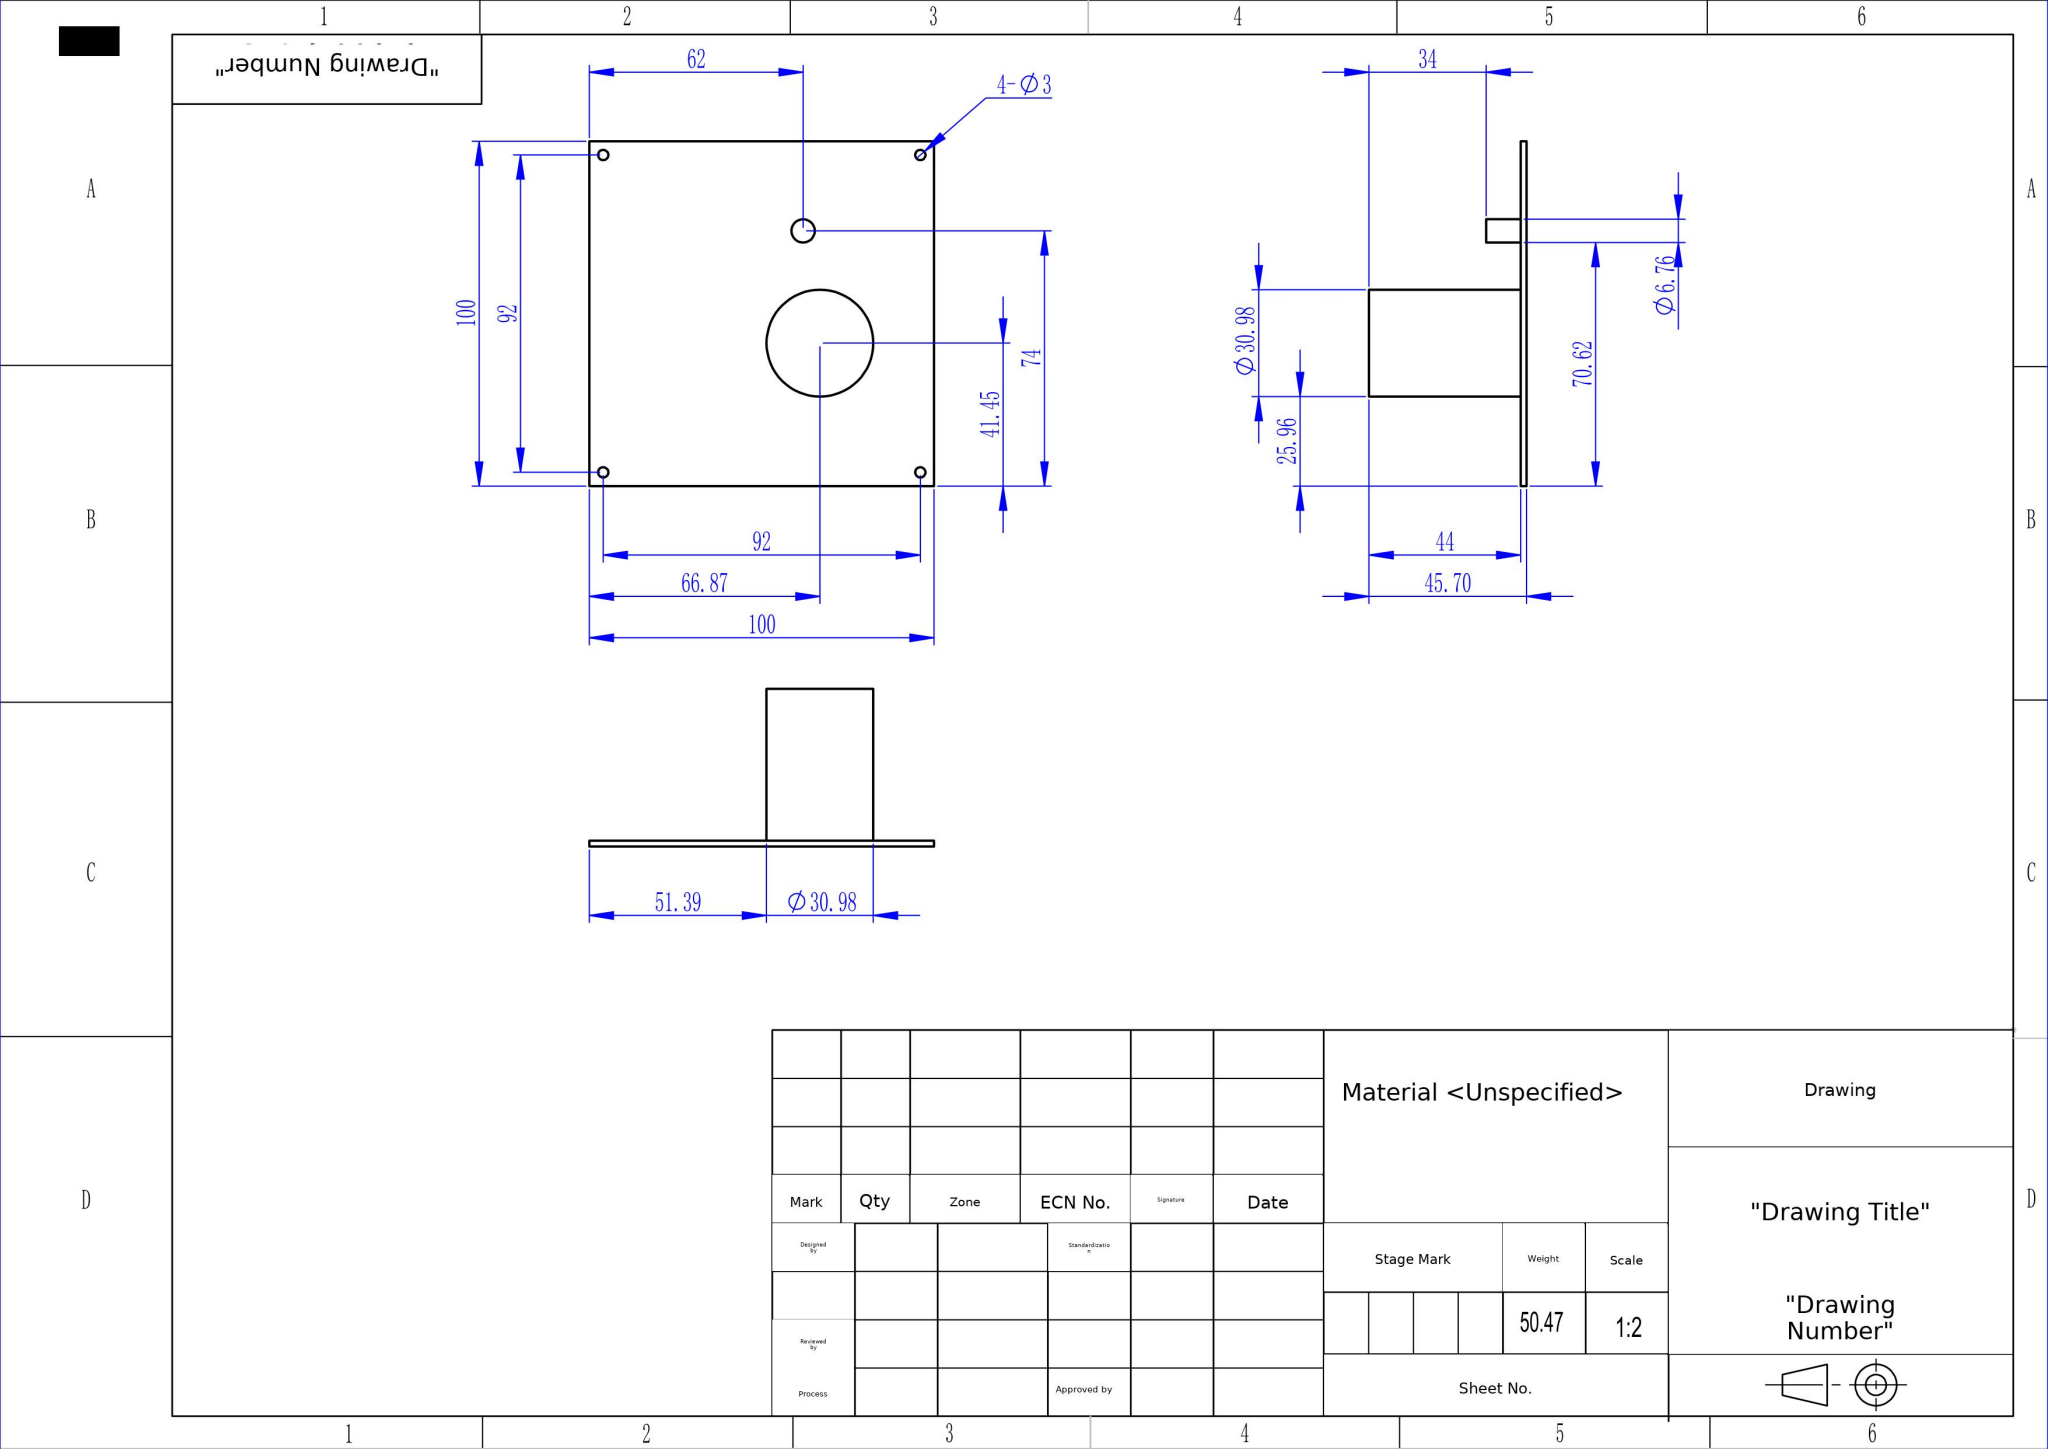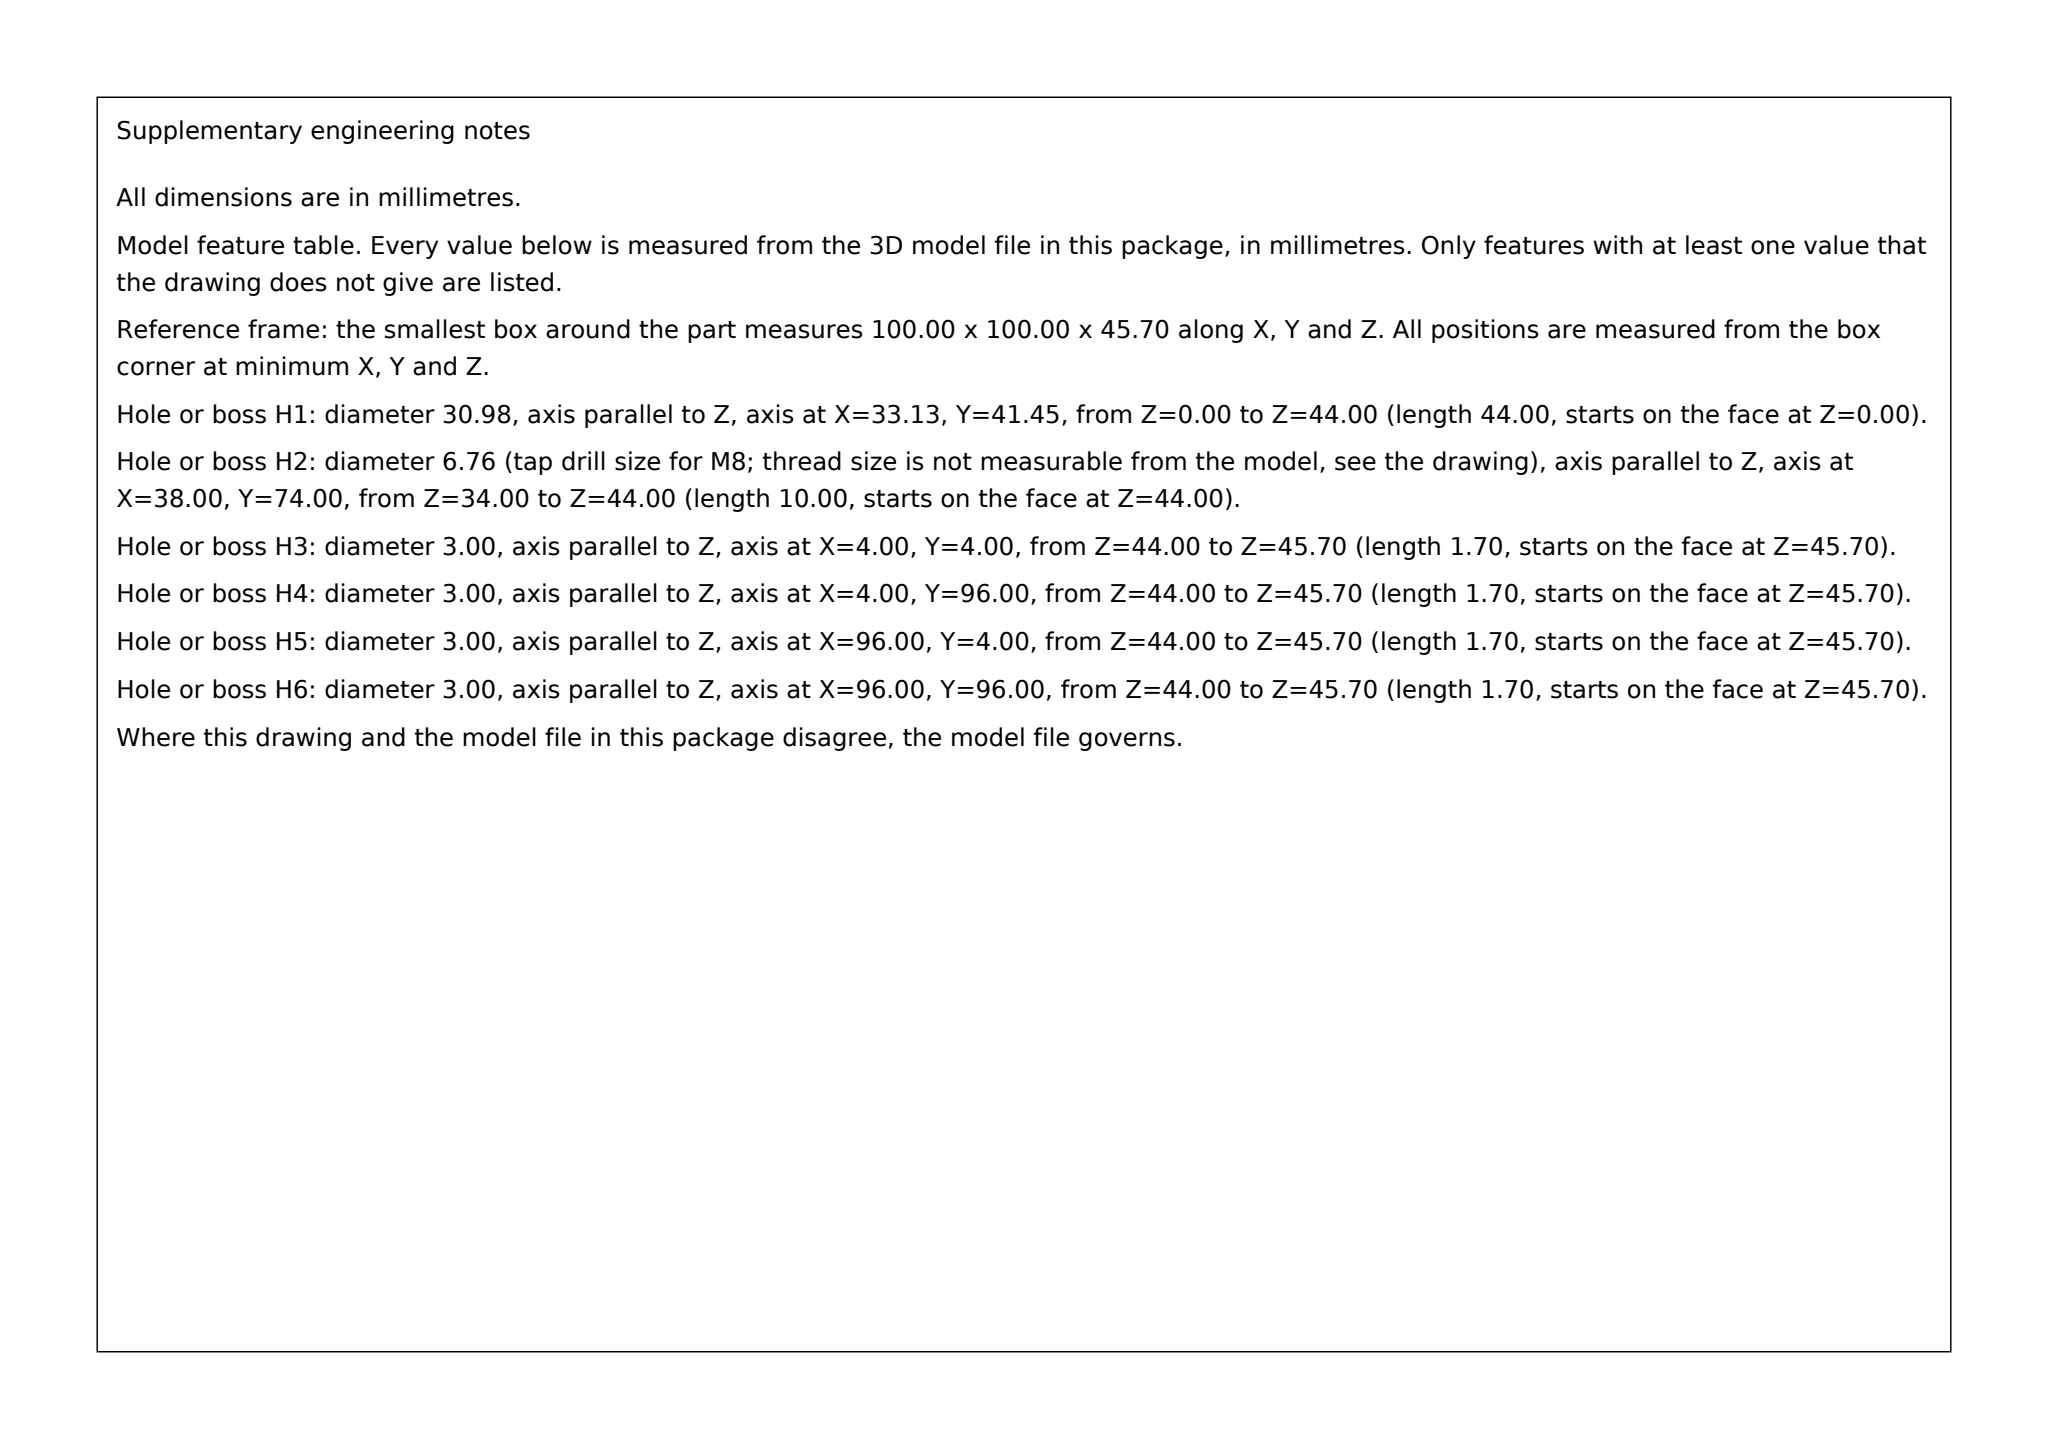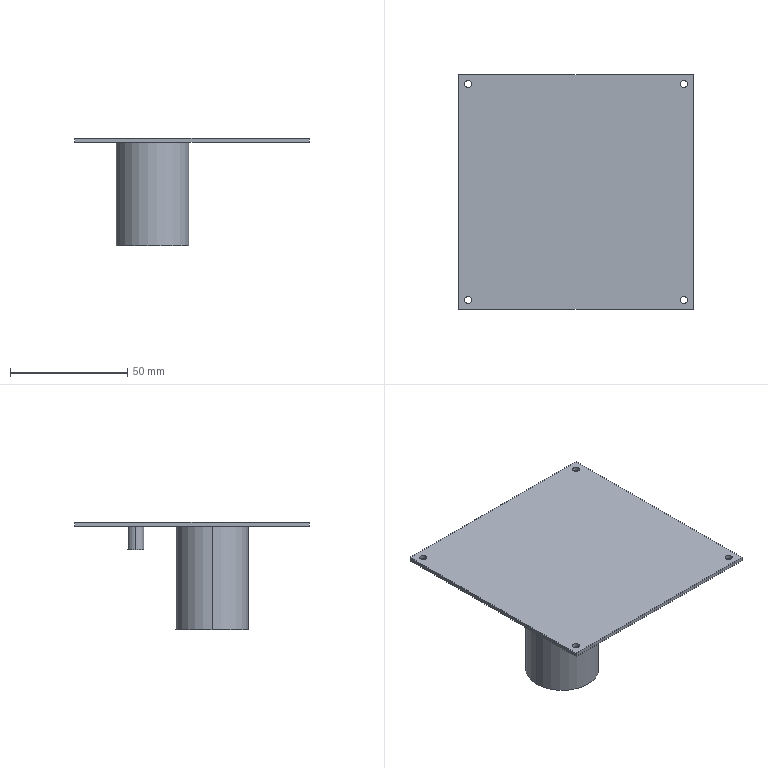Part | SolidWorks | mm | 1 solid | 20 faces | box 100 x 100 x 45.7 mm | volume 50474 mm3 | cylinder 12 | plane 8 | commonest cylinder face diameters 3 x8 6.758 x2 30.978 x2
build123d program:
from build123d import *

# Parameters (mm, degrees)
SKETCH1_W           = 100
SKETCH1_H           = 100
SKETCH1_R           = 1.5
BOSS_EXTRUDE1_DEPTH = 1.7
SKETCH3_R           = 15.489
BOSS_EXTRUDE3_DEPTH = 44
SKETCH5_R           = 3.379
BOSS_EXTRUDE4_DEPTH = 10


with BuildPart() as part:
    # Sketch1 → Boss-Extrude1 (new body)
    with BuildSketch(Plane.XY):
        Rectangle(SKETCH1_W, SKETCH1_H)
        with Locations((46, -46)):
            Circle(SKETCH1_R, mode=Mode.SUBTRACT)
        with Locations((46, 46)):
            Circle(SKETCH1_R, mode=Mode.SUBTRACT)
        with Locations((-46, 46)):
            Circle(SKETCH1_R, mode=Mode.SUBTRACT)
        with Locations((-46, -46)):
            Circle(SKETCH1_R, mode=Mode.SUBTRACT)
    extrude(amount=BOSS_EXTRUDE1_DEPTH)

    # Sketch3 → Boss-Extrude3 (add)
    with BuildSketch(Plane(origin=(0, 0, 0), x_dir=(-1, 0, 0), z_dir=(0, 0, -1))):
        with Locations((16.875, -8.549)):
            Circle(SKETCH3_R)
    extrude(amount=BOSS_EXTRUDE3_DEPTH)

    # Sketch5 → Boss-Extrude4 (add)
    with BuildSketch(Plane(origin=(0, 0, 0), x_dir=(-1, 0, 0), z_dir=(0, 0, -1))):
        with Locations((12, 24)):
            Circle(SKETCH5_R)
    extrude(amount=BOSS_EXTRUDE4_DEPTH)


solid = part.part
STEP:
#1=CARTESIAN_POINT('',(-15.379,24.,-10.));
#2=VERTEX_POINT('',#1);
#3=CARTESIAN_POINT('',(-8.621,24.,-10.));
#4=VERTEX_POINT('',#3);
#5=CARTESIAN_POINT('',(-12.,24.,-10.));
#6=DIRECTION('',(0.,0.,-1.));
#7=DIRECTION('',(-1.,0.,0.));
#8=AXIS2_PLACEMENT_3D('',#5,#6,#7);
#9=CIRCLE('',#8,3.379);
#10=EDGE_CURVE('',#2,#4,#9,.T.);
#11=ORIENTED_EDGE('',*,*,#10,.F.);
#12=CARTESIAN_POINT('',(-15.379,24.,0.));
#13=VERTEX_POINT('',#12);
#14=CARTESIAN_POINT('',(-15.379,24.,-10.));
#15=DIRECTION('',(0.,0.,1.));
#16=VECTOR('',#15,1000.);
#17=LINE('',#14,#16);
#18=EDGE_CURVE('',#2,#13,#17,.T.);
#19=ORIENTED_EDGE('',*,*,#18,.T.);
#20=CARTESIAN_POINT('',(-8.621,24.,0.));
#21=VERTEX_POINT('',#20);
#22=CARTESIAN_POINT('',(-12.,24.,0.));
#23=DIRECTION('',(0.,0.,-1.));
#24=DIRECTION('',(-1.,0.,0.));
#25=AXIS2_PLACEMENT_3D('',#22,#23,#24);
#26=CIRCLE('',#25,3.379);
#27=EDGE_CURVE('',#13,#21,#26,.T.);
#28=ORIENTED_EDGE('',*,*,#27,.T.);
#29=CARTESIAN_POINT('',(-8.621,24.,-10.));
#30=DIRECTION('',(0.,0.,1.));
#31=VECTOR('',#30,1000.);
#32=LINE('',#29,#31);
#33=EDGE_CURVE('',#4,#21,#32,.T.);
#34=ORIENTED_EDGE('',*,*,#33,.F.);
#35=EDGE_LOOP('',(#11,#19,#28,#34));
#36=FACE_OUTER_BOUND('',#35,.T.);
#37=CARTESIAN_POINT('',(-12.,24.,-10.));
#38=DIRECTION('',(0.,0.,1.));
#39=DIRECTION('',(1.,0.,0.));
#40=AXIS2_PLACEMENT_3D('',#37,#38,#39);
#41=CYLINDRICAL_SURFACE('',#40,3.379);
#42=ADVANCED_FACE('',(#36),#41,.T.);
#43=CARTESIAN_POINT('',(-32.364,-8.549,-44.));
#44=VERTEX_POINT('',#43);
#45=CARTESIAN_POINT('',(-1.386,-8.549,-44.));
#46=VERTEX_POINT('',#45);
#47=CARTESIAN_POINT('',(-16.875,-8.549,-44.));
#48=DIRECTION('',(0.,0.,-1.));
#49=DIRECTION('',(-1.,0.,0.));
#50=AXIS2_PLACEMENT_3D('',#47,#48,#49);
#51=CIRCLE('',#50,15.489);
#52=EDGE_CURVE('',#44,#46,#51,.T.);
#53=ORIENTED_EDGE('',*,*,#52,.F.);
#54=CARTESIAN_POINT('',(-32.364,-8.549,0.));
#55=VERTEX_POINT('',#54);
#56=CARTESIAN_POINT('',(-32.364,-8.549,-44.));
#57=DIRECTION('',(0.,0.,1.));
#58=VECTOR('',#57,1000.);
#59=LINE('',#56,#58);
#60=EDGE_CURVE('',#44,#55,#59,.T.);
#61=ORIENTED_EDGE('',*,*,#60,.T.);
#62=CARTESIAN_POINT('',(-1.386,-8.549,0.));
#63=VERTEX_POINT('',#62);
#64=CARTESIAN_POINT('',(-16.875,-8.549,0.));
#65=DIRECTION('',(0.,0.,-1.));
#66=DIRECTION('',(-1.,0.,0.));
#67=AXIS2_PLACEMENT_3D('',#64,#65,#66);
#68=CIRCLE('',#67,15.489);
#69=EDGE_CURVE('',#55,#63,#68,.T.);
#70=ORIENTED_EDGE('',*,*,#69,.T.);
#71=CARTESIAN_POINT('',(-1.386,-8.549,-44.));
#72=DIRECTION('',(0.,0.,1.));
#73=VECTOR('',#72,1000.);
#74=LINE('',#71,#73);
#75=EDGE_CURVE('',#46,#63,#74,.T.);
#76=ORIENTED_EDGE('',*,*,#75,.F.);
#77=EDGE_LOOP('',(#53,#61,#70,#76));
#78=FACE_OUTER_BOUND('',#77,.T.);
#79=CARTESIAN_POINT('',(-16.875,-8.549,-44.));
#80=DIRECTION('',(0.,0.,1.));
#81=DIRECTION('',(1.,0.,0.));
#82=AXIS2_PLACEMENT_3D('',#79,#80,#81);
#83=CYLINDRICAL_SURFACE('',#82,15.489);
#84=ADVANCED_FACE('',(#78),#83,.T.);
#85=CARTESIAN_POINT('',(-47.5,-46.,1.7));
#86=VERTEX_POINT('',#85);
#87=CARTESIAN_POINT('',(-44.5,-46.,1.7));
#88=VERTEX_POINT('',#87);
#89=CARTESIAN_POINT('',(-46.,-46.,1.7));
#90=DIRECTION('',(0.,0.,1.));
#91=DIRECTION('',(1.,0.,0.));
#92=AXIS2_PLACEMENT_3D('',#89,#90,#91);
#93=CIRCLE('',#92,1.5);
#94=EDGE_CURVE('',#86,#88,#93,.T.);
#95=ORIENTED_EDGE('',*,*,#94,.T.);
#96=CARTESIAN_POINT('',(-44.5,-46.,0.));
#97=VERTEX_POINT('',#96);
#98=CARTESIAN_POINT('',(-44.5,-46.,1.7));
#99=DIRECTION('',(0.,0.,-1.));
#100=VECTOR('',#99,1000.);
#101=LINE('',#98,#100);
#102=EDGE_CURVE('',#88,#97,#101,.T.);
#103=ORIENTED_EDGE('',*,*,#102,.T.);
#104=CARTESIAN_POINT('',(-47.5,-46.,0.));
#105=VERTEX_POINT('',#104);
#106=CARTESIAN_POINT('',(-46.,-46.,0.));
#107=DIRECTION('',(0.,0.,1.));
#108=DIRECTION('',(1.,0.,0.));
#109=AXIS2_PLACEMENT_3D('',#106,#107,#108);
#110=CIRCLE('',#109,1.5);
#111=EDGE_CURVE('',#105,#97,#110,.T.);
#112=ORIENTED_EDGE('',*,*,#111,.F.);
#113=CARTESIAN_POINT('',(-47.5,-46.,1.7));
#114=DIRECTION('',(0.,0.,-1.));
#115=VECTOR('',#114,1000.);
#116=LINE('',#113,#115);
#117=EDGE_CURVE('',#86,#105,#116,.T.);
#118=ORIENTED_EDGE('',*,*,#117,.F.);
#119=EDGE_LOOP('',(#95,#103,#112,#118));
#120=FACE_OUTER_BOUND('',#119,.T.);
#121=CARTESIAN_POINT('',(-46.,-46.,1.7));
#122=DIRECTION('',(0.,0.,-1.));
#123=DIRECTION('',(-1.,0.,0.));
#124=AXIS2_PLACEMENT_3D('',#121,#122,#123);
#125=CYLINDRICAL_SURFACE('',#124,1.5);
#126=ADVANCED_FACE('',(#120),#125,.F.);
#127=CARTESIAN_POINT('',(-47.5,46.,1.7));
#128=VERTEX_POINT('',#127);
#129=CARTESIAN_POINT('',(-44.5,46.,1.7));
#130=VERTEX_POINT('',#129);
#131=CARTESIAN_POINT('',(-46.,46.,1.7));
#132=DIRECTION('',(0.,0.,1.));
#133=DIRECTION('',(1.,0.,0.));
#134=AXIS2_PLACEMENT_3D('',#131,#132,#133);
#135=CIRCLE('',#134,1.5);
#136=EDGE_CURVE('',#128,#130,#135,.T.);
#137=ORIENTED_EDGE('',*,*,#136,.T.);
#138=CARTESIAN_POINT('',(-44.5,46.,0.));
#139=VERTEX_POINT('',#138);
#140=CARTESIAN_POINT('',(-44.5,46.,1.7));
#141=DIRECTION('',(0.,0.,-1.));
#142=VECTOR('',#141,1000.);
#143=LINE('',#140,#142);
#144=EDGE_CURVE('',#130,#139,#143,.T.);
#145=ORIENTED_EDGE('',*,*,#144,.T.);
#146=CARTESIAN_POINT('',(-47.5,46.,0.));
#147=VERTEX_POINT('',#146);
#148=CARTESIAN_POINT('',(-46.,46.,0.));
#149=DIRECTION('',(0.,0.,1.));
#150=DIRECTION('',(1.,0.,0.));
#151=AXIS2_PLACEMENT_3D('',#148,#149,#150);
#152=CIRCLE('',#151,1.5);
#153=EDGE_CURVE('',#147,#139,#152,.T.);
#154=ORIENTED_EDGE('',*,*,#153,.F.);
#155=CARTESIAN_POINT('',(-47.5,46.,1.7));
#156=DIRECTION('',(0.,0.,-1.));
#157=VECTOR('',#156,1000.);
#158=LINE('',#155,#157);
#159=EDGE_CURVE('',#128,#147,#158,.T.);
#160=ORIENTED_EDGE('',*,*,#159,.F.);
#161=EDGE_LOOP('',(#137,#145,#154,#160));
#162=FACE_OUTER_BOUND('',#161,.T.);
#163=CARTESIAN_POINT('',(-46.,46.,1.7));
#164=DIRECTION('',(0.,0.,-1.));
#165=DIRECTION('',(-1.,0.,0.));
#166=AXIS2_PLACEMENT_3D('',#163,#164,#165);
#167=CYLINDRICAL_SURFACE('',#166,1.5);
#168=ADVANCED_FACE('',(#162),#167,.F.);
#169=CARTESIAN_POINT('',(44.5,46.,1.7));
#170=VERTEX_POINT('',#169);
#171=CARTESIAN_POINT('',(47.5,46.,1.7));
#172=VERTEX_POINT('',#171);
#173=CARTESIAN_POINT('',(46.,46.,1.7));
#174=DIRECTION('',(0.,0.,1.));
#175=DIRECTION('',(1.,0.,0.));
#176=AXIS2_PLACEMENT_3D('',#173,#174,#175);
#177=CIRCLE('',#176,1.5);
#178=EDGE_CURVE('',#170,#172,#177,.T.);
#179=ORIENTED_EDGE('',*,*,#178,.T.);
#180=CARTESIAN_POINT('',(47.5,46.,0.));
#181=VERTEX_POINT('',#180);
#182=CARTESIAN_POINT('',(47.5,46.,1.7));
#183=DIRECTION('',(0.,0.,-1.));
#184=VECTOR('',#183,1000.);
#185=LINE('',#182,#184);
#186=EDGE_CURVE('',#172,#181,#185,.T.);
#187=ORIENTED_EDGE('',*,*,#186,.T.);
#188=CARTESIAN_POINT('',(44.5,46.,0.));
#189=VERTEX_POINT('',#188);
#190=CARTESIAN_POINT('',(46.,46.,0.));
#191=DIRECTION('',(0.,0.,1.));
#192=DIRECTION('',(1.,0.,0.));
#193=AXIS2_PLACEMENT_3D('',#190,#191,#192);
#194=CIRCLE('',#193,1.5);
#195=EDGE_CURVE('',#189,#181,#194,.T.);
#196=ORIENTED_EDGE('',*,*,#195,.F.);
#197=CARTESIAN_POINT('',(44.5,46.,1.7));
#198=DIRECTION('',(0.,0.,-1.));
#199=VECTOR('',#198,1000.);
#200=LINE('',#197,#199);
#201=EDGE_CURVE('',#170,#189,#200,.T.);
#202=ORIENTED_EDGE('',*,*,#201,.F.);
#203=EDGE_LOOP('',(#179,#187,#196,#202));
#204=FACE_OUTER_BOUND('',#203,.T.);
#205=CARTESIAN_POINT('',(46.,46.,1.7));
#206=DIRECTION('',(0.,0.,-1.));
#207=DIRECTION('',(-1.,0.,0.));
#208=AXIS2_PLACEMENT_3D('',#205,#206,#207);
#209=CYLINDRICAL_SURFACE('',#208,1.5);
#210=ADVANCED_FACE('',(#204),#209,.F.);
#211=CARTESIAN_POINT('',(44.5,-46.,1.7));
#212=VERTEX_POINT('',#211);
#213=CARTESIAN_POINT('',(47.5,-46.,1.7));
#214=VERTEX_POINT('',#213);
#215=CARTESIAN_POINT('',(46.,-46.,1.7));
#216=DIRECTION('',(0.,0.,1.));
#217=DIRECTION('',(1.,0.,0.));
#218=AXIS2_PLACEMENT_3D('',#215,#216,#217);
#219=CIRCLE('',#218,1.5);
#220=EDGE_CURVE('',#212,#214,#219,.T.);
#221=ORIENTED_EDGE('',*,*,#220,.T.);
#222=CARTESIAN_POINT('',(47.5,-46.,0.));
#223=VERTEX_POINT('',#222);
#224=CARTESIAN_POINT('',(47.5,-46.,1.7));
#225=DIRECTION('',(0.,0.,-1.));
#226=VECTOR('',#225,1000.);
#227=LINE('',#224,#226);
#228=EDGE_CURVE('',#214,#223,#227,.T.);
#229=ORIENTED_EDGE('',*,*,#228,.T.);
#230=CARTESIAN_POINT('',(44.5,-46.,0.));
#231=VERTEX_POINT('',#230);
#232=CARTESIAN_POINT('',(46.,-46.,0.));
#233=DIRECTION('',(0.,0.,1.));
#234=DIRECTION('',(1.,0.,0.));
#235=AXIS2_PLACEMENT_3D('',#232,#233,#234);
#236=CIRCLE('',#235,1.5);
#237=EDGE_CURVE('',#231,#223,#236,.T.);
#238=ORIENTED_EDGE('',*,*,#237,.F.);
#239=CARTESIAN_POINT('',(44.5,-46.,1.7));
#240=DIRECTION('',(0.,0.,-1.));
#241=VECTOR('',#240,1000.);
#242=LINE('',#239,#241);
#243=EDGE_CURVE('',#212,#231,#242,.T.);
#244=ORIENTED_EDGE('',*,*,#243,.F.);
#245=EDGE_LOOP('',(#221,#229,#238,#244));
#246=FACE_OUTER_BOUND('',#245,.T.);
#247=CARTESIAN_POINT('',(46.,-46.,1.7));
#248=DIRECTION('',(0.,0.,-1.));
#249=DIRECTION('',(-1.,0.,0.));
#250=AXIS2_PLACEMENT_3D('',#247,#248,#249);
#251=CYLINDRICAL_SURFACE('',#250,1.5);
#252=ADVANCED_FACE('',(#246),#251,.F.);
#253=CARTESIAN_POINT('',(50.,-50.,1.7));
#254=VERTEX_POINT('',#253);
#255=CARTESIAN_POINT('',(50.,50.,1.7));
#256=VERTEX_POINT('',#255);
#257=CARTESIAN_POINT('',(50.,-50.,1.7));
#258=DIRECTION('',(0.,1.,0.));
#259=VECTOR('',#258,1000.);
#260=LINE('',#257,#259);
#261=EDGE_CURVE('',#254,#256,#260,.T.);
#262=ORIENTED_EDGE('',*,*,#261,.T.);
#263=CARTESIAN_POINT('',(-50.,50.,1.7));
#264=VERTEX_POINT('',#263);
#265=CARTESIAN_POINT('',(-50.,50.,1.7));
#266=DIRECTION('',(-1.,0.,0.));
#267=VECTOR('',#266,1000.);
#268=LINE('',#265,#267);
#269=EDGE_CURVE('',#256,#264,#268,.T.);
#270=ORIENTED_EDGE('',*,*,#269,.T.);
#271=CARTESIAN_POINT('',(-50.,-50.,1.7));
#272=VERTEX_POINT('',#271);
#273=CARTESIAN_POINT('',(-50.,-50.,1.7));
#274=DIRECTION('',(0.,-1.,0.));
#275=VECTOR('',#274,1000.);
#276=LINE('',#273,#275);
#277=EDGE_CURVE('',#264,#272,#276,.T.);
#278=ORIENTED_EDGE('',*,*,#277,.T.);
#279=CARTESIAN_POINT('',(-50.,-50.,1.7));
#280=DIRECTION('',(1.,0.,0.));
#281=VECTOR('',#280,1000.);
#282=LINE('',#279,#281);
#283=EDGE_CURVE('',#272,#254,#282,.T.);
#284=ORIENTED_EDGE('',*,*,#283,.T.);
#285=EDGE_LOOP('',(#262,#270,#278,#284));
#286=FACE_OUTER_BOUND('',#285,.T.);
#287=ORIENTED_EDGE('',*,*,#220,.F.);
#288=CARTESIAN_POINT('',(46.,-46.,1.7));
#289=DIRECTION('',(0.,0.,1.));
#290=DIRECTION('',(1.,0.,0.));
#291=AXIS2_PLACEMENT_3D('',#288,#289,#290);
#292=CIRCLE('',#291,1.5);
#293=EDGE_CURVE('',#214,#212,#292,.T.);
#294=ORIENTED_EDGE('',*,*,#293,.F.);
#295=EDGE_LOOP('',(#287,#294));
#296=FACE_BOUND('',#295,.T.);
#297=ORIENTED_EDGE('',*,*,#178,.F.);
#298=CARTESIAN_POINT('',(46.,46.,1.7));
#299=DIRECTION('',(0.,0.,1.));
#300=DIRECTION('',(1.,0.,0.));
#301=AXIS2_PLACEMENT_3D('',#298,#299,#300);
#302=CIRCLE('',#301,1.5);
#303=EDGE_CURVE('',#172,#170,#302,.T.);
#304=ORIENTED_EDGE('',*,*,#303,.F.);
#305=EDGE_LOOP('',(#297,#304));
#306=FACE_BOUND('',#305,.T.);
#307=ORIENTED_EDGE('',*,*,#136,.F.);
#308=CARTESIAN_POINT('',(-46.,46.,1.7));
#309=DIRECTION('',(0.,0.,1.));
#310=DIRECTION('',(1.,0.,0.));
#311=AXIS2_PLACEMENT_3D('',#308,#309,#310);
#312=CIRCLE('',#311,1.5);
#313=EDGE_CURVE('',#130,#128,#312,.T.);
#314=ORIENTED_EDGE('',*,*,#313,.F.);
#315=EDGE_LOOP('',(#307,#314));
#316=FACE_BOUND('',#315,.T.);
#317=ORIENTED_EDGE('',*,*,#94,.F.);
#318=CARTESIAN_POINT('',(-46.,-46.,1.7));
#319=DIRECTION('',(0.,0.,1.));
#320=DIRECTION('',(1.,0.,0.));
#321=AXIS2_PLACEMENT_3D('',#318,#319,#320);
#322=CIRCLE('',#321,1.5);
#323=EDGE_CURVE('',#88,#86,#322,.T.);
#324=ORIENTED_EDGE('',*,*,#323,.F.);
#325=EDGE_LOOP('',(#317,#324));
#326=FACE_BOUND('',#325,.T.);
#327=CARTESIAN_POINT('',(0.,0.,1.7));
#328=DIRECTION('',(0.,0.,-1.));
#329=DIRECTION('',(-1.,0.,0.));
#330=AXIS2_PLACEMENT_3D('',#327,#328,#329);
#331=PLANE('',#330);
#332=ADVANCED_FACE('',(#286,#296,#306,#316,#326),#331,.F.);
#333=CARTESIAN_POINT('',(-12.,24.,0.));
#334=DIRECTION('',(0.,0.,-1.));
#335=DIRECTION('',(-1.,0.,0.));
#336=AXIS2_PLACEMENT_3D('',#333,#334,#335);
#337=CIRCLE('',#336,3.379);
#338=EDGE_CURVE('',#21,#13,#337,.T.);
#339=ORIENTED_EDGE('',*,*,#338,.F.);
#340=ORIENTED_EDGE('',*,*,#27,.F.);
#341=EDGE_LOOP('',(#339,#340));
#342=FACE_BOUND('',#341,.T.);
#343=CARTESIAN_POINT('',(-16.875,-8.549,0.));
#344=DIRECTION('',(0.,0.,-1.));
#345=DIRECTION('',(-1.,0.,0.));
#346=AXIS2_PLACEMENT_3D('',#343,#344,#345);
#347=CIRCLE('',#346,15.489);
#348=EDGE_CURVE('',#63,#55,#347,.T.);
#349=ORIENTED_EDGE('',*,*,#348,.F.);
#350=ORIENTED_EDGE('',*,*,#69,.F.);
#351=EDGE_LOOP('',(#349,#350));
#352=FACE_BOUND('',#351,.T.);
#353=ORIENTED_EDGE('',*,*,#153,.T.);
#354=CARTESIAN_POINT('',(-46.,46.,0.));
#355=DIRECTION('',(0.,0.,1.));
#356=DIRECTION('',(1.,0.,0.));
#357=AXIS2_PLACEMENT_3D('',#354,#355,#356);
#358=CIRCLE('',#357,1.5);
#359=EDGE_CURVE('',#139,#147,#358,.T.);
#360=ORIENTED_EDGE('',*,*,#359,.T.);
#361=EDGE_LOOP('',(#353,#360));
#362=FACE_BOUND('',#361,.T.);
#363=ORIENTED_EDGE('',*,*,#237,.T.);
#364=CARTESIAN_POINT('',(46.,-46.,0.));
#365=DIRECTION('',(0.,0.,1.));
#366=DIRECTION('',(1.,0.,0.));
#367=AXIS2_PLACEMENT_3D('',#364,#365,#366);
#368=CIRCLE('',#367,1.5);
#369=EDGE_CURVE('',#223,#231,#368,.T.);
#370=ORIENTED_EDGE('',*,*,#369,.T.);
#371=EDGE_LOOP('',(#363,#370));
#372=FACE_BOUND('',#371,.T.);
#373=CARTESIAN_POINT('',(50.,-50.,0.));
#374=VERTEX_POINT('',#373);
#375=CARTESIAN_POINT('',(50.,50.,0.));
#376=VERTEX_POINT('',#375);
#377=CARTESIAN_POINT('',(50.,-50.,0.));
#378=DIRECTION('',(0.,1.,0.));
#379=VECTOR('',#378,1000.);
#380=LINE('',#377,#379);
#381=EDGE_CURVE('',#374,#376,#380,.T.);
#382=ORIENTED_EDGE('',*,*,#381,.F.);
#383=CARTESIAN_POINT('',(-50.,-50.,0.));
#384=VERTEX_POINT('',#383);
#385=CARTESIAN_POINT('',(-50.,-50.,0.));
#386=DIRECTION('',(1.,0.,0.));
#387=VECTOR('',#386,1000.);
#388=LINE('',#385,#387);
#389=EDGE_CURVE('',#384,#374,#388,.T.);
#390=ORIENTED_EDGE('',*,*,#389,.F.);
#391=CARTESIAN_POINT('',(-50.,50.,0.));
#392=VERTEX_POINT('',#391);
#393=CARTESIAN_POINT('',(-50.,-50.,0.));
#394=DIRECTION('',(0.,-1.,0.));
#395=VECTOR('',#394,1000.);
#396=LINE('',#393,#395);
#397=EDGE_CURVE('',#392,#384,#396,.T.);
#398=ORIENTED_EDGE('',*,*,#397,.F.);
#399=CARTESIAN_POINT('',(-50.,50.,0.));
#400=DIRECTION('',(-1.,0.,0.));
#401=VECTOR('',#400,1000.);
#402=LINE('',#399,#401);
#403=EDGE_CURVE('',#376,#392,#402,.T.);
#404=ORIENTED_EDGE('',*,*,#403,.F.);
#405=EDGE_LOOP('',(#382,#390,#398,#404));
#406=FACE_OUTER_BOUND('',#405,.T.);
#407=ORIENTED_EDGE('',*,*,#195,.T.);
#408=CARTESIAN_POINT('',(46.,46.,0.));
#409=DIRECTION('',(0.,0.,1.));
#410=DIRECTION('',(1.,0.,0.));
#411=AXIS2_PLACEMENT_3D('',#408,#409,#410);
#412=CIRCLE('',#411,1.5);
#413=EDGE_CURVE('',#181,#189,#412,.T.);
#414=ORIENTED_EDGE('',*,*,#413,.T.);
#415=EDGE_LOOP('',(#407,#414));
#416=FACE_BOUND('',#415,.T.);
#417=ORIENTED_EDGE('',*,*,#111,.T.);
#418=CARTESIAN_POINT('',(-46.,-46.,0.));
#419=DIRECTION('',(0.,0.,1.));
#420=DIRECTION('',(1.,0.,0.));
#421=AXIS2_PLACEMENT_3D('',#418,#419,#420);
#422=CIRCLE('',#421,1.5);
#423=EDGE_CURVE('',#97,#105,#422,.T.);
#424=ORIENTED_EDGE('',*,*,#423,.T.);
#425=EDGE_LOOP('',(#417,#424));
#426=FACE_BOUND('',#425,.T.);
#427=CARTESIAN_POINT('',(0.,0.,0.));
#428=DIRECTION('',(0.,0.,-1.));
#429=DIRECTION('',(-1.,0.,0.));
#430=AXIS2_PLACEMENT_3D('',#427,#428,#429);
#431=PLANE('',#430);
#432=ADVANCED_FACE('',(#342,#352,#362,#372,#406,#416,#426),#431,.T.);
#433=ORIENTED_EDGE('',*,*,#381,.T.);
#434=CARTESIAN_POINT('',(50.,50.,1.7));
#435=DIRECTION('',(0.,0.,-1.));
#436=VECTOR('',#435,1000.);
#437=LINE('',#434,#436);
#438=EDGE_CURVE('',#256,#376,#437,.T.);
#439=ORIENTED_EDGE('',*,*,#438,.F.);
#440=ORIENTED_EDGE('',*,*,#261,.F.);
#441=CARTESIAN_POINT('',(50.,-50.,1.7));
#442=DIRECTION('',(0.,0.,-1.));
#443=VECTOR('',#442,1000.);
#444=LINE('',#441,#443);
#445=EDGE_CURVE('',#254,#374,#444,.T.);
#446=ORIENTED_EDGE('',*,*,#445,.T.);
#447=EDGE_LOOP('',(#433,#439,#440,#446));
#448=FACE_OUTER_BOUND('',#447,.T.);
#449=CARTESIAN_POINT('',(50.,-50.,1.7));
#450=DIRECTION('',(-1.,0.,0.));
#451=DIRECTION('',(0.,0.,1.));
#452=AXIS2_PLACEMENT_3D('',#449,#450,#451);
#453=PLANE('',#452);
#454=ADVANCED_FACE('',(#448),#453,.F.);
#455=ORIENTED_EDGE('',*,*,#403,.T.);
#456=CARTESIAN_POINT('',(-50.,50.,1.7));
#457=DIRECTION('',(0.,0.,-1.));
#458=VECTOR('',#457,1000.);
#459=LINE('',#456,#458);
#460=EDGE_CURVE('',#264,#392,#459,.T.);
#461=ORIENTED_EDGE('',*,*,#460,.F.);
#462=ORIENTED_EDGE('',*,*,#269,.F.);
#463=ORIENTED_EDGE('',*,*,#438,.T.);
#464=EDGE_LOOP('',(#455,#461,#462,#463));
#465=FACE_OUTER_BOUND('',#464,.T.);
#466=CARTESIAN_POINT('',(-50.,50.,1.7));
#467=DIRECTION('',(0.,-1.,0.));
#468=DIRECTION('',(0.,0.,-1.));
#469=AXIS2_PLACEMENT_3D('',#466,#467,#468);
#470=PLANE('',#469);
#471=ADVANCED_FACE('',(#465),#470,.F.);
#472=ORIENTED_EDGE('',*,*,#397,.T.);
#473=CARTESIAN_POINT('',(-50.,-50.,1.7));
#474=DIRECTION('',(0.,0.,-1.));
#475=VECTOR('',#474,1000.);
#476=LINE('',#473,#475);
#477=EDGE_CURVE('',#272,#384,#476,.T.);
#478=ORIENTED_EDGE('',*,*,#477,.F.);
#479=ORIENTED_EDGE('',*,*,#277,.F.);
#480=ORIENTED_EDGE('',*,*,#460,.T.);
#481=EDGE_LOOP('',(#472,#478,#479,#480));
#482=FACE_OUTER_BOUND('',#481,.T.);
#483=CARTESIAN_POINT('',(-50.,-50.,1.7));
#484=DIRECTION('',(1.,0.,0.));
#485=DIRECTION('',(0.,0.,-1.));
#486=AXIS2_PLACEMENT_3D('',#483,#484,#485);
#487=PLANE('',#486);
#488=ADVANCED_FACE('',(#482),#487,.F.);
#489=ORIENTED_EDGE('',*,*,#389,.T.);
#490=ORIENTED_EDGE('',*,*,#445,.F.);
#491=ORIENTED_EDGE('',*,*,#283,.F.);
#492=ORIENTED_EDGE('',*,*,#477,.T.);
#493=EDGE_LOOP('',(#489,#490,#491,#492));
#494=FACE_OUTER_BOUND('',#493,.T.);
#495=CARTESIAN_POINT('',(-50.,-50.,1.7));
#496=DIRECTION('',(0.,1.,0.));
#497=DIRECTION('',(0.,0.,1.));
#498=AXIS2_PLACEMENT_3D('',#495,#496,#497);
#499=PLANE('',#498);
#500=ADVANCED_FACE('',(#494),#499,.F.);
#501=ORIENTED_EDGE('',*,*,#228,.F.);
#502=ORIENTED_EDGE('',*,*,#293,.T.);
#503=ORIENTED_EDGE('',*,*,#243,.T.);
#504=ORIENTED_EDGE('',*,*,#369,.F.);
#505=EDGE_LOOP('',(#501,#502,#503,#504));
#506=FACE_OUTER_BOUND('',#505,.T.);
#507=CARTESIAN_POINT('',(46.,-46.,1.7));
#508=DIRECTION('',(0.,0.,-1.));
#509=DIRECTION('',(-1.,0.,0.));
#510=AXIS2_PLACEMENT_3D('',#507,#508,#509);
#511=CYLINDRICAL_SURFACE('',#510,1.5);
#512=ADVANCED_FACE('',(#506),#511,.F.);
#513=ORIENTED_EDGE('',*,*,#186,.F.);
#514=ORIENTED_EDGE('',*,*,#303,.T.);
#515=ORIENTED_EDGE('',*,*,#201,.T.);
#516=ORIENTED_EDGE('',*,*,#413,.F.);
#517=EDGE_LOOP('',(#513,#514,#515,#516));
#518=FACE_OUTER_BOUND('',#517,.T.);
#519=CARTESIAN_POINT('',(46.,46.,1.7));
#520=DIRECTION('',(0.,0.,-1.));
#521=DIRECTION('',(-1.,0.,0.));
#522=AXIS2_PLACEMENT_3D('',#519,#520,#521);
#523=CYLINDRICAL_SURFACE('',#522,1.5);
#524=ADVANCED_FACE('',(#518),#523,.F.);
#525=ORIENTED_EDGE('',*,*,#144,.F.);
#526=ORIENTED_EDGE('',*,*,#313,.T.);
#527=ORIENTED_EDGE('',*,*,#159,.T.);
#528=ORIENTED_EDGE('',*,*,#359,.F.);
#529=EDGE_LOOP('',(#525,#526,#527,#528));
#530=FACE_OUTER_BOUND('',#529,.T.);
#531=CARTESIAN_POINT('',(-46.,46.,1.7));
#532=DIRECTION('',(0.,0.,-1.));
#533=DIRECTION('',(-1.,0.,0.));
#534=AXIS2_PLACEMENT_3D('',#531,#532,#533);
#535=CYLINDRICAL_SURFACE('',#534,1.5);
#536=ADVANCED_FACE('',(#530),#535,.F.);
#537=ORIENTED_EDGE('',*,*,#102,.F.);
#538=ORIENTED_EDGE('',*,*,#323,.T.);
#539=ORIENTED_EDGE('',*,*,#117,.T.);
#540=ORIENTED_EDGE('',*,*,#423,.F.);
#541=EDGE_LOOP('',(#537,#538,#539,#540));
#542=FACE_OUTER_BOUND('',#541,.T.);
#543=CARTESIAN_POINT('',(-46.,-46.,1.7));
#544=DIRECTION('',(0.,0.,-1.));
#545=DIRECTION('',(-1.,0.,0.));
#546=AXIS2_PLACEMENT_3D('',#543,#544,#545);
#547=CYLINDRICAL_SURFACE('',#546,1.5);
#548=ADVANCED_FACE('',(#542),#547,.F.);
#549=ORIENTED_EDGE('',*,*,#60,.F.);
#550=CARTESIAN_POINT('',(-16.875,-8.549,-44.));
#551=DIRECTION('',(0.,0.,-1.));
#552=DIRECTION('',(-1.,0.,0.));
#553=AXIS2_PLACEMENT_3D('',#550,#551,#552);
#554=CIRCLE('',#553,15.489);
#555=EDGE_CURVE('',#46,#44,#554,.T.);
#556=ORIENTED_EDGE('',*,*,#555,.F.);
#557=ORIENTED_EDGE('',*,*,#75,.T.);
#558=ORIENTED_EDGE('',*,*,#348,.T.);
#559=EDGE_LOOP('',(#549,#556,#557,#558));
#560=FACE_OUTER_BOUND('',#559,.T.);
#561=CARTESIAN_POINT('',(-16.875,-8.549,-44.));
#562=DIRECTION('',(0.,0.,1.));
#563=DIRECTION('',(1.,0.,0.));
#564=AXIS2_PLACEMENT_3D('',#561,#562,#563);
#565=CYLINDRICAL_SURFACE('',#564,15.489);
#566=ADVANCED_FACE('',(#560),#565,.T.);
#567=ORIENTED_EDGE('',*,*,#555,.T.);
#568=ORIENTED_EDGE('',*,*,#52,.T.);
#569=EDGE_LOOP('',(#567,#568));
#570=FACE_OUTER_BOUND('',#569,.T.);
#571=CARTESIAN_POINT('',(-16.875,-8.549,-44.));
#572=DIRECTION('',(0.,0.,-1.));
#573=DIRECTION('',(-1.,0.,0.));
#574=AXIS2_PLACEMENT_3D('',#571,#572,#573);
#575=PLANE('',#574);
#576=ADVANCED_FACE('',(#570),#575,.T.);
#577=ORIENTED_EDGE('',*,*,#18,.F.);
#578=CARTESIAN_POINT('',(-12.,24.,-10.));
#579=DIRECTION('',(0.,0.,-1.));
#580=DIRECTION('',(-1.,0.,0.));
#581=AXIS2_PLACEMENT_3D('',#578,#579,#580);
#582=CIRCLE('',#581,3.379);
#583=EDGE_CURVE('',#4,#2,#582,.T.);
#584=ORIENTED_EDGE('',*,*,#583,.F.);
#585=ORIENTED_EDGE('',*,*,#33,.T.);
#586=ORIENTED_EDGE('',*,*,#338,.T.);
#587=EDGE_LOOP('',(#577,#584,#585,#586));
#588=FACE_OUTER_BOUND('',#587,.T.);
#589=CARTESIAN_POINT('',(-12.,24.,-10.));
#590=DIRECTION('',(0.,0.,1.));
#591=DIRECTION('',(1.,0.,0.));
#592=AXIS2_PLACEMENT_3D('',#589,#590,#591);
#593=CYLINDRICAL_SURFACE('',#592,3.379);
#594=ADVANCED_FACE('',(#588),#593,.T.);
#595=ORIENTED_EDGE('',*,*,#583,.T.);
#596=ORIENTED_EDGE('',*,*,#10,.T.);
#597=EDGE_LOOP('',(#595,#596));
#598=FACE_OUTER_BOUND('',#597,.T.);
#599=CARTESIAN_POINT('',(-12.,24.,-10.));
#600=DIRECTION('',(0.,0.,-1.));
#601=DIRECTION('',(-1.,0.,0.));
#602=AXIS2_PLACEMENT_3D('',#599,#600,#601);
#603=PLANE('',#602);
#604=ADVANCED_FACE('',(#598),#603,.T.);
#605=CLOSED_SHELL('',(#42,#84,#126,#168,#210,#252,#332,#432,#454,#471,#488,#500,#512,#524,#536,#548,#566,#576,#594,#604));
#606=MANIFOLD_SOLID_BREP('',#605);
#607=CARTESIAN_POINT('',(0.,0.,0.));
#608=DIRECTION('',(0.,0.,1.));
#609=DIRECTION('',(1.,0.,0.));
#610=AXIS2_PLACEMENT_3D('',#607,#608,#609);
#611=(LENGTH_UNIT()NAMED_UNIT(*)SI_UNIT(.MILLI.,.METRE.));
#612=UNCERTAINTY_MEASURE_WITH_UNIT(LENGTH_MEASURE(0.00001),#611,'','');
#613=(NAMED_UNIT(*)PLANE_ANGLE_UNIT()SI_UNIT($,.RADIAN.));
#614=(NAMED_UNIT(*)SI_UNIT($,.STERADIAN.)SOLID_ANGLE_UNIT());
#615=(GEOMETRIC_REPRESENTATION_CONTEXT(3)GLOBAL_UNCERTAINTY_ASSIGNED_CONTEXT((#612))GLOBAL_UNIT_ASSIGNED_CONTEXT((#611,#613,#614))REPRESENTATION_CONTEXT('',''));
#616=ADVANCED_BREP_SHAPE_REPRESENTATION('',(#606,#610),#615);